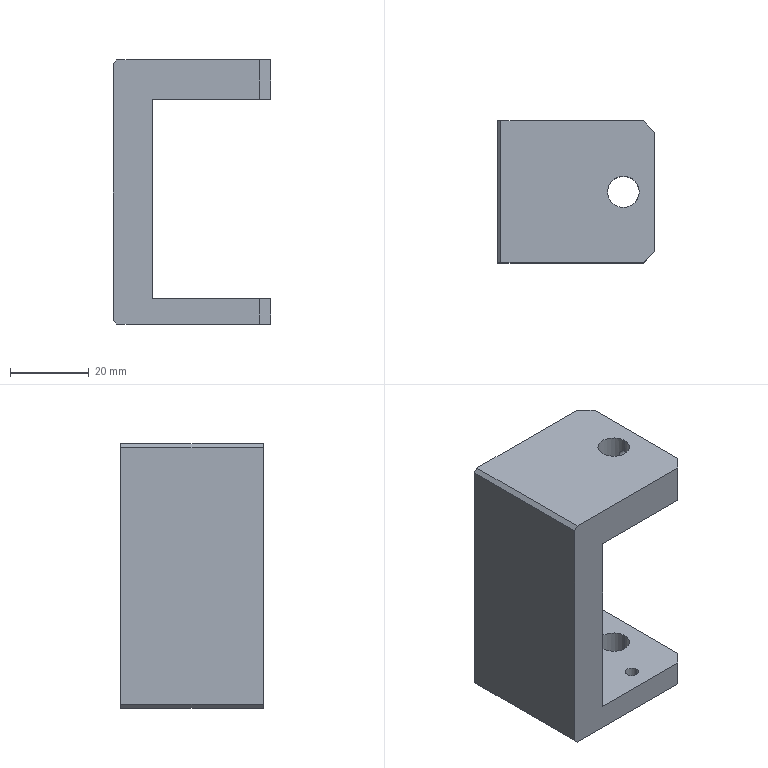Component | SolidWorks | 170423A4-ConveyorBeltIdlerAssembly1-1_170423A4-ConveyorBeltIdlerFixture1-1 | 1 solid | 34 faces | box 40 x 36 x 67 mm | volume 40578 mm3 | plane 16 | cylinder 14 | cone 4 | commonest cylinder face diameters 3.3 x10 8 x4
STEP:
#1=CARTESIAN_POINT('',(0.7383,-3.771,18.844));
#2=VERTEX_POINT('',#1);
#3=CARTESIAN_POINT('',(0.7383,-3.771,18.715));
#4=VERTEX_POINT('',#3);
#5=CARTESIAN_POINT('',(0.7383,-3.771,18.844));
#6=CARTESIAN_POINT('',(0.7383,-3.775,18.844));
#7=CARTESIAN_POINT('',(0.7382,-3.78,18.844));
#8=CARTESIAN_POINT('',(0.7375,-3.788,18.842));
#9=CARTESIAN_POINT('',(0.737,-3.792,18.841));
#10=CARTESIAN_POINT('',(0.7351,-3.804,18.836));
#11=CARTESIAN_POINT('',(0.7333,-3.811,18.831));
#12=CARTESIAN_POINT('',(0.7306,-3.82,18.822));
#13=CARTESIAN_POINT('',(0.7297,-3.823,18.819));
#14=CARTESIAN_POINT('',(0.7279,-3.827,18.812));
#15=CARTESIAN_POINT('',(0.7271,-3.83,18.808));
#16=CARTESIAN_POINT('',(0.7258,-3.833,18.801));
#17=CARTESIAN_POINT('',(0.7253,-3.834,18.797));
#18=CARTESIAN_POINT('',(0.7245,-3.836,18.788));
#19=CARTESIAN_POINT('',(0.7243,-3.836,18.784));
#20=CARTESIAN_POINT('',(0.7243,-3.836,18.771));
#21=CARTESIAN_POINT('',(0.7251,-3.834,18.762));
#22=CARTESIAN_POINT('',(0.7271,-3.83,18.751));
#23=CARTESIAN_POINT('',(0.7279,-3.827,18.747));
#24=CARTESIAN_POINT('',(0.7297,-3.823,18.74));
#25=CARTESIAN_POINT('',(0.7306,-3.82,18.737));
#26=CARTESIAN_POINT('',(0.7324,-3.814,18.731));
#27=CARTESIAN_POINT('',(0.7333,-3.811,18.728));
#28=CARTESIAN_POINT('',(0.7349,-3.804,18.723));
#29=CARTESIAN_POINT('',(0.7357,-3.8,18.721));
#30=CARTESIAN_POINT('',(0.7376,-3.788,18.716));
#31=CARTESIAN_POINT('',(0.7383,-3.78,18.715));
#32=CARTESIAN_POINT('',(0.7383,-3.771,18.715));
#33=B_SPLINE_CURVE_WITH_KNOTS('',3,(#5,#6,#7,#8,#9,#10,#11,#12,#13,#14,#15,#16,#17,#18,#19,#20,#21,#22,#23,#24,#25,#26,#27,#28,#29,#30,#31,#32),.UNSPECIFIED.,.F.,.F.,(4,2,2,2,2,2,2,2,2,2,2,2,2,4),(0.005218,0.005543,0.005869,0.006521,0.006847,0.007173,0.007499,0.007824,0.008476,0.008802,0.009128,0.009454,0.009779,0.01043),.UNSPECIFIED.);
#34=EDGE_CURVE('',#2,#4,#33,.T.);
#35=ORIENTED_EDGE('',*,*,#34,.F.);
#36=CARTESIAN_POINT('',(0.8958,-3.771,18.844));
#37=VERTEX_POINT('',#36);
#38=CARTESIAN_POINT('',(0.8958,-3.771,18.844));
#39=DIRECTION('',(1.,0.,0.));
#40=VECTOR('',#39,39.37);
#41=LINE('',#38,#40);
#42=EDGE_CURVE('',#2,#37,#41,.T.);
#43=ORIENTED_EDGE('',*,*,#42,.T.);
#44=CARTESIAN_POINT('',(0.8958,-3.771,18.715));
#45=VERTEX_POINT('',#44);
#46=CARTESIAN_POINT('',(0.8958,-3.771,18.78));
#47=DIRECTION('',(1.,0.,0.));
#48=DIRECTION('',(0.,0.,-1.));
#49=AXIS2_PLACEMENT_3D('',#46,#47,#48);
#50=CIRCLE('',#49,0.06496);
#51=EDGE_CURVE('',#37,#45,#50,.T.);
#52=ORIENTED_EDGE('',*,*,#51,.T.);
#53=CARTESIAN_POINT('',(0.8958,-3.771,18.715));
#54=DIRECTION('',(1.,0.,0.));
#55=VECTOR('',#54,39.37);
#56=LINE('',#53,#55);
#57=EDGE_CURVE('',#4,#45,#56,.T.);
#58=ORIENTED_EDGE('',*,*,#57,.F.);
#59=EDGE_LOOP('',(#35,#43,#52,#58));
#60=FACE_OUTER_BOUND('',#59,.T.);
#61=CARTESIAN_POINT('',(0.8958,-3.771,18.78));
#62=DIRECTION('',(1.,0.,0.));
#63=DIRECTION('',(0.,0.,-1.));
#64=AXIS2_PLACEMENT_3D('',#61,#62,#63);
#65=CYLINDRICAL_SURFACE('',#64,0.06496);
#66=ADVANCED_FACE('',(#60),#65,.F.);
#67=CARTESIAN_POINT('',(0.2797,-3.279,16.594));
#68=VERTEX_POINT('',#67);
#69=CARTESIAN_POINT('',(0.4096,-3.279,16.594));
#70=VERTEX_POINT('',#69);
#71=CARTESIAN_POINT('',(0.3446,-3.279,16.594));
#72=DIRECTION('',(0.,0.,1.));
#73=DIRECTION('',(-1.,0.,0.));
#74=AXIS2_PLACEMENT_3D('',#71,#72,#73);
#75=CIRCLE('',#74,0.06496);
#76=EDGE_CURVE('',#68,#70,#75,.T.);
#77=ORIENTED_EDGE('',*,*,#76,.T.);
#78=CARTESIAN_POINT('',(0.4096,-3.279,16.339));
#79=VERTEX_POINT('',#78);
#80=CARTESIAN_POINT('',(0.4096,-3.279,16.339));
#81=DIRECTION('',(0.,0.,-1.));
#82=VECTOR('',#81,39.37);
#83=LINE('',#80,#82);
#84=EDGE_CURVE('',#70,#79,#83,.T.);
#85=ORIENTED_EDGE('',*,*,#84,.T.);
#86=CARTESIAN_POINT('',(0.2797,-3.279,16.339));
#87=VERTEX_POINT('',#86);
#88=CARTESIAN_POINT('',(0.3446,-3.279,16.339));
#89=DIRECTION('',(0.,0.,-1.));
#90=DIRECTION('',(-1.,0.,0.));
#91=AXIS2_PLACEMENT_3D('',#88,#89,#90);
#92=CIRCLE('',#91,0.06496);
#93=EDGE_CURVE('',#79,#87,#92,.T.);
#94=ORIENTED_EDGE('',*,*,#93,.T.);
#95=CARTESIAN_POINT('',(0.2797,-3.279,16.339));
#96=DIRECTION('',(0.,0.,-1.));
#97=VECTOR('',#96,39.37);
#98=LINE('',#95,#97);
#99=EDGE_CURVE('',#68,#87,#98,.T.);
#100=ORIENTED_EDGE('',*,*,#99,.F.);
#101=EDGE_LOOP('',(#77,#85,#94,#100));
#102=FACE_OUTER_BOUND('',#101,.T.);
#103=CARTESIAN_POINT('',(0.3446,-3.279,16.339));
#104=DIRECTION('',(0.,0.,-1.));
#105=DIRECTION('',(-1.,0.,0.));
#106=AXIS2_PLACEMENT_3D('',#103,#104,#105);
#107=CYLINDRICAL_SURFACE('',#106,0.06496);
#108=ADVANCED_FACE('',(#102),#107,.F.);
#109=CARTESIAN_POINT('',(0.2797,-4.263,16.594));
#110=VERTEX_POINT('',#109);
#111=CARTESIAN_POINT('',(0.4096,-4.263,16.594));
#112=VERTEX_POINT('',#111);
#113=CARTESIAN_POINT('',(0.3446,-4.263,16.594));
#114=DIRECTION('',(0.,0.,1.));
#115=DIRECTION('',(-1.,0.,0.));
#116=AXIS2_PLACEMENT_3D('',#113,#114,#115);
#117=CIRCLE('',#116,0.06496);
#118=EDGE_CURVE('',#110,#112,#117,.T.);
#119=ORIENTED_EDGE('',*,*,#118,.T.);
#120=CARTESIAN_POINT('',(0.4096,-4.263,16.339));
#121=VERTEX_POINT('',#120);
#122=CARTESIAN_POINT('',(0.4096,-4.263,16.339));
#123=DIRECTION('',(0.,0.,-1.));
#124=VECTOR('',#123,39.37);
#125=LINE('',#122,#124);
#126=EDGE_CURVE('',#112,#121,#125,.T.);
#127=ORIENTED_EDGE('',*,*,#126,.T.);
#128=CARTESIAN_POINT('',(0.2797,-4.263,16.339));
#129=VERTEX_POINT('',#128);
#130=CARTESIAN_POINT('',(0.3446,-4.263,16.339));
#131=DIRECTION('',(0.,0.,-1.));
#132=DIRECTION('',(-1.,0.,0.));
#133=AXIS2_PLACEMENT_3D('',#130,#131,#132);
#134=CIRCLE('',#133,0.06496);
#135=EDGE_CURVE('',#121,#129,#134,.T.);
#136=ORIENTED_EDGE('',*,*,#135,.T.);
#137=CARTESIAN_POINT('',(0.2797,-4.263,16.339));
#138=DIRECTION('',(0.,0.,-1.));
#139=VECTOR('',#138,39.37);
#140=LINE('',#137,#139);
#141=EDGE_CURVE('',#110,#129,#140,.T.);
#142=ORIENTED_EDGE('',*,*,#141,.F.);
#143=EDGE_LOOP('',(#119,#127,#136,#142));
#144=FACE_OUTER_BOUND('',#143,.T.);
#145=CARTESIAN_POINT('',(0.3446,-4.263,16.339));
#146=DIRECTION('',(0.,0.,-1.));
#147=DIRECTION('',(-1.,0.,0.));
#148=AXIS2_PLACEMENT_3D('',#145,#146,#147);
#149=CYLINDRICAL_SURFACE('',#148,0.06496);
#150=ADVANCED_FACE('',(#144),#149,.F.);
#151=CARTESIAN_POINT('',(-0.3778,-3.279,16.791));
#152=VERTEX_POINT('',#151);
#153=CARTESIAN_POINT('',(-0.5077,-3.279,16.791));
#154=VERTEX_POINT('',#153);
#155=CARTESIAN_POINT('',(-0.4428,-3.279,16.791));
#156=DIRECTION('',(0.,0.,-1.));
#157=DIRECTION('',(-1.,0.,0.));
#158=AXIS2_PLACEMENT_3D('',#155,#156,#157);
#159=CIRCLE('',#158,0.06496);
#160=EDGE_CURVE('',#152,#154,#159,.T.);
#161=ORIENTED_EDGE('',*,*,#160,.F.);
#162=CARTESIAN_POINT('',(-0.3778,-3.279,16.339));
#163=VERTEX_POINT('',#162);
#164=CARTESIAN_POINT('',(-0.3778,-3.279,16.339));
#165=DIRECTION('',(0.,0.,-1.));
#166=VECTOR('',#165,39.37);
#167=LINE('',#164,#166);
#168=EDGE_CURVE('',#152,#163,#167,.T.);
#169=ORIENTED_EDGE('',*,*,#168,.T.);
#170=CARTESIAN_POINT('',(-0.5077,-3.279,16.339));
#171=VERTEX_POINT('',#170);
#172=CARTESIAN_POINT('',(-0.4428,-3.279,16.339));
#173=DIRECTION('',(0.,0.,-1.));
#174=DIRECTION('',(-1.,0.,0.));
#175=AXIS2_PLACEMENT_3D('',#172,#173,#174);
#176=CIRCLE('',#175,0.06496);
#177=EDGE_CURVE('',#163,#171,#176,.T.);
#178=ORIENTED_EDGE('',*,*,#177,.T.);
#179=CARTESIAN_POINT('',(-0.5077,-3.279,16.339));
#180=DIRECTION('',(0.,0.,-1.));
#181=VECTOR('',#180,39.37);
#182=LINE('',#179,#181);
#183=EDGE_CURVE('',#154,#171,#182,.T.);
#184=ORIENTED_EDGE('',*,*,#183,.F.);
#185=EDGE_LOOP('',(#161,#169,#178,#184));
#186=FACE_OUTER_BOUND('',#185,.T.);
#187=CARTESIAN_POINT('',(-0.4428,-3.279,16.339));
#188=DIRECTION('',(0.,0.,-1.));
#189=DIRECTION('',(-1.,0.,0.));
#190=AXIS2_PLACEMENT_3D('',#187,#188,#189);
#191=CYLINDRICAL_SURFACE('',#190,0.06496);
#192=ADVANCED_FACE('',(#186),#191,.F.);
#193=CARTESIAN_POINT('',(-0.4428,-3.279,16.83));
#194=VERTEX_POINT('',#193);
#195=CARTESIAN_POINT('',(-0.5077,-3.279,16.791));
#196=DIRECTION('',(-0.8572,0.,-0.515));
#197=VECTOR('',#196,39.37);
#198=LINE('',#195,#197);
#199=EDGE_CURVE('',#194,#154,#198,.T.);
#200=ORIENTED_EDGE('',*,*,#199,.F.);
#201=CARTESIAN_POINT('',(-0.3778,-3.279,16.791));
#202=DIRECTION('',(0.8572,0.,-0.515));
#203=VECTOR('',#202,39.37);
#204=LINE('',#201,#203);
#205=EDGE_CURVE('',#194,#152,#204,.T.);
#206=ORIENTED_EDGE('',*,*,#205,.T.);
#207=ORIENTED_EDGE('',*,*,#160,.T.);
#208=EDGE_LOOP('',(#200,#206,#207));
#209=FACE_OUTER_BOUND('',#208,.T.);
#210=CARTESIAN_POINT('',(-0.4428,-3.279,16.791));
#211=DIRECTION('',(0.,0.,-1.));
#212=DIRECTION('',(-1.,0.,0.));
#213=AXIS2_PLACEMENT_3D('',#210,#211,#212);
#214=CONICAL_SURFACE('',#213,0.06496,1.03);
#215=ADVANCED_FACE('',(#209),#214,.F.);
#216=CARTESIAN_POINT('',(-0.3778,-4.263,16.791));
#217=VERTEX_POINT('',#216);
#218=CARTESIAN_POINT('',(-0.5077,-4.263,16.791));
#219=VERTEX_POINT('',#218);
#220=CARTESIAN_POINT('',(-0.4428,-4.263,16.791));
#221=DIRECTION('',(0.,0.,-1.));
#222=DIRECTION('',(-1.,0.,0.));
#223=AXIS2_PLACEMENT_3D('',#220,#221,#222);
#224=CIRCLE('',#223,0.06496);
#225=EDGE_CURVE('',#217,#219,#224,.T.);
#226=ORIENTED_EDGE('',*,*,#225,.F.);
#227=CARTESIAN_POINT('',(-0.3778,-4.263,16.339));
#228=VERTEX_POINT('',#227);
#229=CARTESIAN_POINT('',(-0.3778,-4.263,16.339));
#230=DIRECTION('',(0.,0.,-1.));
#231=VECTOR('',#230,39.37);
#232=LINE('',#229,#231);
#233=EDGE_CURVE('',#217,#228,#232,.T.);
#234=ORIENTED_EDGE('',*,*,#233,.T.);
#235=CARTESIAN_POINT('',(-0.5077,-4.263,16.339));
#236=VERTEX_POINT('',#235);
#237=CARTESIAN_POINT('',(-0.4428,-4.263,16.339));
#238=DIRECTION('',(0.,0.,-1.));
#239=DIRECTION('',(-1.,0.,0.));
#240=AXIS2_PLACEMENT_3D('',#237,#238,#239);
#241=CIRCLE('',#240,0.06496);
#242=EDGE_CURVE('',#228,#236,#241,.T.);
#243=ORIENTED_EDGE('',*,*,#242,.T.);
#244=CARTESIAN_POINT('',(-0.5077,-4.263,16.339));
#245=DIRECTION('',(0.,0.,-1.));
#246=VECTOR('',#245,39.37);
#247=LINE('',#244,#246);
#248=EDGE_CURVE('',#219,#236,#247,.T.);
#249=ORIENTED_EDGE('',*,*,#248,.F.);
#250=EDGE_LOOP('',(#226,#234,#243,#249));
#251=FACE_OUTER_BOUND('',#250,.T.);
#252=CARTESIAN_POINT('',(-0.4428,-4.263,16.339));
#253=DIRECTION('',(0.,0.,-1.));
#254=DIRECTION('',(-1.,0.,0.));
#255=AXIS2_PLACEMENT_3D('',#252,#253,#254);
#256=CYLINDRICAL_SURFACE('',#255,0.06496);
#257=ADVANCED_FACE('',(#251),#256,.F.);
#258=CARTESIAN_POINT('',(-0.4428,-4.263,16.83));
#259=VERTEX_POINT('',#258);
#260=CARTESIAN_POINT('',(-0.5077,-4.263,16.791));
#261=DIRECTION('',(-0.8572,0.,-0.515));
#262=VECTOR('',#261,39.37);
#263=LINE('',#260,#262);
#264=EDGE_CURVE('',#259,#219,#263,.T.);
#265=ORIENTED_EDGE('',*,*,#264,.F.);
#266=CARTESIAN_POINT('',(-0.3778,-4.263,16.791));
#267=DIRECTION('',(0.8572,0.,-0.515));
#268=VECTOR('',#267,39.37);
#269=LINE('',#266,#268);
#270=EDGE_CURVE('',#259,#217,#269,.T.);
#271=ORIENTED_EDGE('',*,*,#270,.T.);
#272=ORIENTED_EDGE('',*,*,#225,.T.);
#273=EDGE_LOOP('',(#265,#271,#272));
#274=FACE_OUTER_BOUND('',#273,.T.);
#275=CARTESIAN_POINT('',(-0.4428,-4.263,16.791));
#276=DIRECTION('',(0.,0.,-1.));
#277=DIRECTION('',(-1.,0.,0.));
#278=AXIS2_PLACEMENT_3D('',#275,#276,#277);
#279=CONICAL_SURFACE('',#278,0.06496,1.03);
#280=ADVANCED_FACE('',(#274),#279,.F.);
#281=CARTESIAN_POINT('',(0.4234,-3.771,16.339));
#282=VERTEX_POINT('',#281);
#283=CARTESIAN_POINT('',(0.7383,-3.771,16.339));
#284=VERTEX_POINT('',#283);
#285=CARTESIAN_POINT('',(0.5808,-3.771,16.339));
#286=DIRECTION('',(0.,0.,1.));
#287=DIRECTION('',(1.,0.,0.));
#288=AXIS2_PLACEMENT_3D('',#285,#286,#287);
#289=CIRCLE('',#288,0.1575);
#290=EDGE_CURVE('',#282,#284,#289,.T.);
#291=ORIENTED_EDGE('',*,*,#290,.F.);
#292=CARTESIAN_POINT('',(0.4234,-3.771,16.594));
#293=VERTEX_POINT('',#292);
#294=CARTESIAN_POINT('',(0.4234,-3.771,18.976));
#295=DIRECTION('',(0.,0.,1.));
#296=VECTOR('',#295,39.37);
#297=LINE('',#294,#296);
#298=EDGE_CURVE('',#282,#293,#297,.T.);
#299=ORIENTED_EDGE('',*,*,#298,.T.);
#300=CARTESIAN_POINT('',(0.7383,-3.771,16.594));
#301=VERTEX_POINT('',#300);
#302=CARTESIAN_POINT('',(0.5808,-3.771,16.594));
#303=DIRECTION('',(0.,0.,1.));
#304=DIRECTION('',(-1.,0.,0.));
#305=AXIS2_PLACEMENT_3D('',#302,#303,#304);
#306=CIRCLE('',#305,0.1575);
#307=EDGE_CURVE('',#293,#301,#306,.T.);
#308=ORIENTED_EDGE('',*,*,#307,.T.);
#309=CARTESIAN_POINT('',(0.7383,-3.771,18.976));
#310=DIRECTION('',(0.,0.,1.));
#311=VECTOR('',#310,39.37);
#312=LINE('',#309,#311);
#313=EDGE_CURVE('',#284,#301,#312,.T.);
#314=ORIENTED_EDGE('',*,*,#313,.F.);
#315=EDGE_LOOP('',(#291,#299,#308,#314));
#316=FACE_OUTER_BOUND('',#315,.T.);
#317=CARTESIAN_POINT('',(0.5808,-3.771,18.976));
#318=DIRECTION('',(0.,0.,1.));
#319=DIRECTION('',(1.,0.,0.));
#320=AXIS2_PLACEMENT_3D('',#317,#318,#319);
#321=CYLINDRICAL_SURFACE('',#320,0.1575);
#322=ADVANCED_FACE('',(#316),#321,.F.);
#323=CARTESIAN_POINT('',(0.7383,-3.771,18.583));
#324=VERTEX_POINT('',#323);
#325=CARTESIAN_POINT('',(0.4234,-3.771,18.583));
#326=VERTEX_POINT('',#325);
#327=CARTESIAN_POINT('',(0.5808,-3.771,18.583));
#328=DIRECTION('',(-0.,0.,-1.));
#329=DIRECTION('',(1.,0.,0.));
#330=AXIS2_PLACEMENT_3D('',#327,#328,#329);
#331=CIRCLE('',#330,0.1575);
#332=EDGE_CURVE('',#324,#326,#331,.T.);
#333=ORIENTED_EDGE('',*,*,#332,.T.);
#334=CARTESIAN_POINT('',(0.4234,-3.771,18.976));
#335=VERTEX_POINT('',#334);
#336=CARTESIAN_POINT('',(0.4234,-3.771,18.976));
#337=DIRECTION('',(0.,0.,1.));
#338=VECTOR('',#337,39.37);
#339=LINE('',#336,#338);
#340=EDGE_CURVE('',#326,#335,#339,.T.);
#341=ORIENTED_EDGE('',*,*,#340,.T.);
#342=CARTESIAN_POINT('',(0.7383,-3.771,18.976));
#343=VERTEX_POINT('',#342);
#344=CARTESIAN_POINT('',(0.5808,-3.771,18.976));
#345=DIRECTION('',(0.,0.,1.));
#346=DIRECTION('',(1.,0.,0.));
#347=AXIS2_PLACEMENT_3D('',#344,#345,#346);
#348=CIRCLE('',#347,0.1575);
#349=EDGE_CURVE('',#335,#343,#348,.T.);
#350=ORIENTED_EDGE('',*,*,#349,.T.);
#351=CARTESIAN_POINT('',(0.7383,-3.771,18.976));
#352=DIRECTION('',(0.,0.,1.));
#353=VECTOR('',#352,39.37);
#354=LINE('',#351,#353);
#355=EDGE_CURVE('',#2,#343,#354,.T.);
#356=ORIENTED_EDGE('',*,*,#355,.F.);
#357=ORIENTED_EDGE('',*,*,#34,.T.);
#358=CARTESIAN_POINT('',(0.7383,-3.771,18.976));
#359=DIRECTION('',(0.,0.,1.));
#360=VECTOR('',#359,39.37);
#361=LINE('',#358,#360);
#362=EDGE_CURVE('',#324,#4,#361,.T.);
#363=ORIENTED_EDGE('',*,*,#362,.F.);
#364=EDGE_LOOP('',(#333,#341,#350,#356,#357,#363));
#365=FACE_OUTER_BOUND('',#364,.T.);
#366=CARTESIAN_POINT('',(0.5808,-3.771,18.976));
#367=DIRECTION('',(0.,0.,1.));
#368=DIRECTION('',(1.,0.,0.));
#369=AXIS2_PLACEMENT_3D('',#366,#367,#368);
#370=CYLINDRICAL_SURFACE('',#369,0.1575);
#371=ADVANCED_FACE('',(#365),#370,.F.);
#372=CARTESIAN_POINT('',(0.8958,-3.771,18.78));
#373=DIRECTION('',(1.,0.,0.));
#374=DIRECTION('',(0.,0.,-1.));
#375=AXIS2_PLACEMENT_3D('',#372,#373,#374);
#376=CIRCLE('',#375,0.06496);
#377=EDGE_CURVE('',#45,#37,#376,.T.);
#378=ORIENTED_EDGE('',*,*,#377,.F.);
#379=ORIENTED_EDGE('',*,*,#51,.F.);
#380=EDGE_LOOP('',(#378,#379));
#381=FACE_BOUND('',#380,.T.);
#382=CARTESIAN_POINT('',(0.8958,-4.362,18.976));
#383=VERTEX_POINT('',#382);
#384=CARTESIAN_POINT('',(0.8958,-3.181,18.976));
#385=VERTEX_POINT('',#384);
#386=CARTESIAN_POINT('',(0.8958,-4.48,18.976));
#387=DIRECTION('',(0.,1.,0.));
#388=VECTOR('',#387,39.37);
#389=LINE('',#386,#388);
#390=EDGE_CURVE('',#383,#385,#389,.T.);
#391=ORIENTED_EDGE('',*,*,#390,.F.);
#392=CARTESIAN_POINT('',(0.8958,-4.362,18.583));
#393=VERTEX_POINT('',#392);
#394=CARTESIAN_POINT('',(0.8958,-4.362,18.976));
#395=DIRECTION('',(0.,0.,-1.));
#396=VECTOR('',#395,39.37);
#397=LINE('',#394,#396);
#398=EDGE_CURVE('',#383,#393,#397,.T.);
#399=ORIENTED_EDGE('',*,*,#398,.T.);
#400=CARTESIAN_POINT('',(0.8958,-3.181,18.583));
#401=VERTEX_POINT('',#400);
#402=CARTESIAN_POINT('',(0.8958,-4.48,18.583));
#403=DIRECTION('',(0.,1.,0.));
#404=VECTOR('',#403,39.37);
#405=LINE('',#402,#404);
#406=EDGE_CURVE('',#393,#401,#405,.T.);
#407=ORIENTED_EDGE('',*,*,#406,.T.);
#408=CARTESIAN_POINT('',(0.8958,-3.181,18.976));
#409=DIRECTION('',(0.,0.,1.));
#410=VECTOR('',#409,39.37);
#411=LINE('',#408,#410);
#412=EDGE_CURVE('',#401,#385,#411,.T.);
#413=ORIENTED_EDGE('',*,*,#412,.T.);
#414=EDGE_LOOP('',(#391,#399,#407,#413));
#415=FACE_OUTER_BOUND('',#414,.T.);
#416=CARTESIAN_POINT('',(0.8958,-4.48,18.976));
#417=DIRECTION('',(-1.,0.,0.));
#418=DIRECTION('',(0.,0.,1.));
#419=AXIS2_PLACEMENT_3D('',#416,#417,#418);
#420=PLANE('',#419);
#421=ADVANCED_FACE('',(#381,#415),#420,.F.);
#422=ORIENTED_EDGE('',*,*,#340,.F.);
#423=CARTESIAN_POINT('',(0.5808,-3.771,18.583));
#424=DIRECTION('',(-0.,0.,-1.));
#425=DIRECTION('',(1.,0.,0.));
#426=AXIS2_PLACEMENT_3D('',#423,#424,#425);
#427=CIRCLE('',#426,0.1575);
#428=EDGE_CURVE('',#326,#324,#427,.T.);
#429=ORIENTED_EDGE('',*,*,#428,.T.);
#430=ORIENTED_EDGE('',*,*,#362,.T.);
#431=CARTESIAN_POINT('',(0.7383,-3.771,18.715));
#432=CARTESIAN_POINT('',(0.7383,-3.767,18.715));
#433=CARTESIAN_POINT('',(0.7382,-3.763,18.715));
#434=CARTESIAN_POINT('',(0.7375,-3.754,18.717));
#435=CARTESIAN_POINT('',(0.737,-3.75,18.718));
#436=CARTESIAN_POINT('',(0.7351,-3.738,18.723));
#437=CARTESIAN_POINT('',(0.7333,-3.731,18.728));
#438=CARTESIAN_POINT('',(0.7297,-3.719,18.74));
#439=CARTESIAN_POINT('',(0.7278,-3.715,18.747));
#440=CARTESIAN_POINT('',(0.7258,-3.71,18.758));
#441=CARTESIAN_POINT('',(0.7252,-3.708,18.763));
#442=CARTESIAN_POINT('',(0.7245,-3.707,18.771));
#443=CARTESIAN_POINT('',(0.7243,-3.706,18.775));
#444=CARTESIAN_POINT('',(0.7243,-3.706,18.784));
#445=CARTESIAN_POINT('',(0.7245,-3.707,18.788));
#446=CARTESIAN_POINT('',(0.7252,-3.708,18.797));
#447=CARTESIAN_POINT('',(0.7258,-3.71,18.801));
#448=CARTESIAN_POINT('',(0.7272,-3.713,18.809));
#449=CARTESIAN_POINT('',(0.7279,-3.715,18.812));
#450=CARTESIAN_POINT('',(0.7297,-3.72,18.819));
#451=CARTESIAN_POINT('',(0.7306,-3.722,18.823));
#452=CARTESIAN_POINT('',(0.7324,-3.728,18.828));
#453=CARTESIAN_POINT('',(0.7333,-3.731,18.831));
#454=CARTESIAN_POINT('',(0.7349,-3.739,18.836));
#455=CARTESIAN_POINT('',(0.7357,-3.742,18.838));
#456=CARTESIAN_POINT('',(0.7376,-3.754,18.843));
#457=CARTESIAN_POINT('',(0.7383,-3.763,18.844));
#458=CARTESIAN_POINT('',(0.7383,-3.771,18.844));
#459=B_SPLINE_CURVE_WITH_KNOTS('',3,(#431,#432,#433,#434,#435,#436,#437,#438,#439,#440,#441,#442,#443,#444,#445,#446,#447,#448,#449,#450,#451,#452,#453,#454,#455,#456,#457,#458),.UNSPECIFIED.,.F.,.F.,(4,2,2,2,2,2,2,2,2,2,2,2,2,4),(0.,0.0003261,0.0006522,0.001304,0.001957,0.002283,0.002609,0.002935,0.003261,0.003587,0.003913,0.004239,0.004565,0.005218),.UNSPECIFIED.);
#460=EDGE_CURVE('',#4,#2,#459,.T.);
#461=ORIENTED_EDGE('',*,*,#460,.T.);
#462=ORIENTED_EDGE('',*,*,#355,.T.);
#463=CARTESIAN_POINT('',(0.5808,-3.771,18.976));
#464=DIRECTION('',(0.,0.,1.));
#465=DIRECTION('',(1.,0.,0.));
#466=AXIS2_PLACEMENT_3D('',#463,#464,#465);
#467=CIRCLE('',#466,0.1575);
#468=EDGE_CURVE('',#343,#335,#467,.T.);
#469=ORIENTED_EDGE('',*,*,#468,.T.);
#470=EDGE_LOOP('',(#422,#429,#430,#461,#462,#469));
#471=FACE_OUTER_BOUND('',#470,.T.);
#472=CARTESIAN_POINT('',(0.5808,-3.771,18.976));
#473=DIRECTION('',(0.,0.,1.));
#474=DIRECTION('',(1.,0.,0.));
#475=AXIS2_PLACEMENT_3D('',#472,#473,#474);
#476=CYLINDRICAL_SURFACE('',#475,0.1575);
#477=ADVANCED_FACE('',(#471),#476,.F.);
#478=CARTESIAN_POINT('',(-0.679,-3.063,18.937));
#479=VERTEX_POINT('',#478);
#480=CARTESIAN_POINT('',(-0.679,-3.063,16.378));
#481=VERTEX_POINT('',#480);
#482=CARTESIAN_POINT('',(-0.679,-3.063,18.976));
#483=DIRECTION('',(0.,0.,-1.));
#484=VECTOR('',#483,39.37);
#485=LINE('',#482,#484);
#486=EDGE_CURVE('',#479,#481,#485,.T.);
#487=ORIENTED_EDGE('',*,*,#486,.T.);
#488=CARTESIAN_POINT('',(-0.679,-4.48,16.378));
#489=VERTEX_POINT('',#488);
#490=CARTESIAN_POINT('',(-0.679,-4.48,16.378));
#491=DIRECTION('',(0.,-1.,0.));
#492=VECTOR('',#491,39.37);
#493=LINE('',#490,#492);
#494=EDGE_CURVE('',#481,#489,#493,.T.);
#495=ORIENTED_EDGE('',*,*,#494,.T.);
#496=CARTESIAN_POINT('',(-0.679,-4.48,18.937));
#497=VERTEX_POINT('',#496);
#498=CARTESIAN_POINT('',(-0.679,-4.48,18.976));
#499=DIRECTION('',(0.,0.,-1.));
#500=VECTOR('',#499,39.37);
#501=LINE('',#498,#500);
#502=EDGE_CURVE('',#497,#489,#501,.T.);
#503=ORIENTED_EDGE('',*,*,#502,.F.);
#504=CARTESIAN_POINT('',(-0.679,-4.48,18.937));
#505=DIRECTION('',(0.,1.,0.));
#506=VECTOR('',#505,39.37);
#507=LINE('',#504,#506);
#508=EDGE_CURVE('',#497,#479,#507,.T.);
#509=ORIENTED_EDGE('',*,*,#508,.T.);
#510=EDGE_LOOP('',(#487,#495,#503,#509));
#511=FACE_OUTER_BOUND('',#510,.T.);
#512=CARTESIAN_POINT('',(-0.679,-4.48,18.976));
#513=DIRECTION('',(1.,0.,0.));
#514=DIRECTION('',(0.,0.,-1.));
#515=AXIS2_PLACEMENT_3D('',#512,#513,#514);
#516=PLANE('',#515);
#517=ADVANCED_FACE('',(#511),#516,.F.);
#518=ORIENTED_EDGE('',*,*,#502,.T.);
#519=CARTESIAN_POINT('',(-0.6396,-4.48,16.339));
#520=VERTEX_POINT('',#519);
#521=CARTESIAN_POINT('',(-0.679,-4.48,16.378));
#522=DIRECTION('',(0.7071,0.,-0.7071));
#523=VECTOR('',#522,39.37);
#524=LINE('',#521,#523);
#525=EDGE_CURVE('',#489,#520,#524,.T.);
#526=ORIENTED_EDGE('',*,*,#525,.T.);
#527=CARTESIAN_POINT('',(0.7777,-4.48,16.339));
#528=VERTEX_POINT('',#527);
#529=CARTESIAN_POINT('',(-0.679,-4.48,16.339));
#530=DIRECTION('',(1.,0.,0.));
#531=VECTOR('',#530,39.37);
#532=LINE('',#529,#531);
#533=EDGE_CURVE('',#520,#528,#532,.T.);
#534=ORIENTED_EDGE('',*,*,#533,.T.);
#535=CARTESIAN_POINT('',(0.7777,-4.48,16.594));
#536=VERTEX_POINT('',#535);
#537=CARTESIAN_POINT('',(0.7777,-4.48,18.976));
#538=DIRECTION('',(0.,0.,1.));
#539=VECTOR('',#538,39.37);
#540=LINE('',#537,#539);
#541=EDGE_CURVE('',#528,#536,#540,.T.);
#542=ORIENTED_EDGE('',*,*,#541,.T.);
#543=CARTESIAN_POINT('',(-0.2853,-4.48,16.594));
#544=VERTEX_POINT('',#543);
#545=CARTESIAN_POINT('',(0.8958,-4.48,16.594));
#546=DIRECTION('',(-1.,0.,0.));
#547=VECTOR('',#546,39.37);
#548=LINE('',#545,#547);
#549=EDGE_CURVE('',#536,#544,#548,.T.);
#550=ORIENTED_EDGE('',*,*,#549,.T.);
#551=CARTESIAN_POINT('',(-0.2853,-4.48,18.583));
#552=VERTEX_POINT('',#551);
#553=CARTESIAN_POINT('',(-0.2853,-4.48,16.594));
#554=DIRECTION('',(0.,0.,1.));
#555=VECTOR('',#554,39.37);
#556=LINE('',#553,#555);
#557=EDGE_CURVE('',#544,#552,#556,.T.);
#558=ORIENTED_EDGE('',*,*,#557,.T.);
#559=CARTESIAN_POINT('',(0.7777,-4.48,18.583));
#560=VERTEX_POINT('',#559);
#561=CARTESIAN_POINT('',(0.8958,-4.48,18.583));
#562=DIRECTION('',(1.,0.,-0.));
#563=VECTOR('',#562,39.37);
#564=LINE('',#561,#563);
#565=EDGE_CURVE('',#552,#560,#564,.T.);
#566=ORIENTED_EDGE('',*,*,#565,.T.);
#567=CARTESIAN_POINT('',(0.7777,-4.48,18.976));
#568=VERTEX_POINT('',#567);
#569=CARTESIAN_POINT('',(0.7777,-4.48,18.976));
#570=DIRECTION('',(0.,0.,1.));
#571=VECTOR('',#570,39.37);
#572=LINE('',#569,#571);
#573=EDGE_CURVE('',#560,#568,#572,.T.);
#574=ORIENTED_EDGE('',*,*,#573,.T.);
#575=CARTESIAN_POINT('',(-0.6396,-4.48,18.976));
#576=VERTEX_POINT('',#575);
#577=CARTESIAN_POINT('',(-0.679,-4.48,18.976));
#578=DIRECTION('',(1.,0.,0.));
#579=VECTOR('',#578,39.37);
#580=LINE('',#577,#579);
#581=EDGE_CURVE('',#576,#568,#580,.T.);
#582=ORIENTED_EDGE('',*,*,#581,.F.);
#583=CARTESIAN_POINT('',(-0.6396,-4.48,18.976));
#584=DIRECTION('',(-0.7071,0.,-0.7071));
#585=VECTOR('',#584,39.37);
#586=LINE('',#583,#585);
#587=EDGE_CURVE('',#576,#497,#586,.T.);
#588=ORIENTED_EDGE('',*,*,#587,.T.);
#589=EDGE_LOOP('',(#518,#526,#534,#542,#550,#558,#566,#574,#582,#588));
#590=FACE_OUTER_BOUND('',#589,.T.);
#591=CARTESIAN_POINT('',(-0.679,-4.48,18.976));
#592=DIRECTION('',(0.,1.,0.));
#593=DIRECTION('',(0.,0.,1.));
#594=AXIS2_PLACEMENT_3D('',#591,#592,#593);
#595=PLANE('',#594);
#596=ADVANCED_FACE('',(#590),#595,.F.);
#597=CARTESIAN_POINT('',(0.8958,-4.362,16.339));
#598=VERTEX_POINT('',#597);
#599=CARTESIAN_POINT('',(0.8958,-3.181,16.339));
#600=VERTEX_POINT('',#599);
#601=CARTESIAN_POINT('',(0.8958,-4.48,16.339));
#602=DIRECTION('',(0.,1.,0.));
#603=VECTOR('',#602,39.37);
#604=LINE('',#601,#603);
#605=EDGE_CURVE('',#598,#600,#604,.T.);
#606=ORIENTED_EDGE('',*,*,#605,.T.);
#607=CARTESIAN_POINT('',(0.8958,-3.181,16.594));
#608=VERTEX_POINT('',#607);
#609=CARTESIAN_POINT('',(0.8958,-3.181,18.976));
#610=DIRECTION('',(0.,0.,1.));
#611=VECTOR('',#610,39.37);
#612=LINE('',#609,#611);
#613=EDGE_CURVE('',#600,#608,#612,.T.);
#614=ORIENTED_EDGE('',*,*,#613,.T.);
#615=CARTESIAN_POINT('',(0.8958,-4.362,16.594));
#616=VERTEX_POINT('',#615);
#617=CARTESIAN_POINT('',(0.8958,-4.48,16.594));
#618=DIRECTION('',(0.,1.,0.));
#619=VECTOR('',#618,39.37);
#620=LINE('',#617,#619);
#621=EDGE_CURVE('',#616,#608,#620,.T.);
#622=ORIENTED_EDGE('',*,*,#621,.F.);
#623=CARTESIAN_POINT('',(0.8958,-4.362,18.976));
#624=DIRECTION('',(0.,0.,-1.));
#625=VECTOR('',#624,39.37);
#626=LINE('',#623,#625);
#627=EDGE_CURVE('',#616,#598,#626,.T.);
#628=ORIENTED_EDGE('',*,*,#627,.T.);
#629=EDGE_LOOP('',(#606,#614,#622,#628));
#630=FACE_OUTER_BOUND('',#629,.T.);
#631=CARTESIAN_POINT('',(0.8958,-4.48,18.976));
#632=DIRECTION('',(-1.,0.,0.));
#633=DIRECTION('',(0.,0.,1.));
#634=AXIS2_PLACEMENT_3D('',#631,#632,#633);
#635=PLANE('',#634);
#636=ADVANCED_FACE('',(#630),#635,.F.);
#637=CARTESIAN_POINT('',(0.7777,-3.063,16.339));
#638=VERTEX_POINT('',#637);
#639=CARTESIAN_POINT('',(-0.6396,-3.063,16.339));
#640=VERTEX_POINT('',#639);
#641=CARTESIAN_POINT('',(-0.679,-3.063,16.339));
#642=DIRECTION('',(-1.,0.,0.));
#643=VECTOR('',#642,39.37);
#644=LINE('',#641,#643);
#645=EDGE_CURVE('',#638,#640,#644,.T.);
#646=ORIENTED_EDGE('',*,*,#645,.T.);
#647=CARTESIAN_POINT('',(-0.679,-3.063,16.378));
#648=DIRECTION('',(-0.7071,0.,0.7071));
#649=VECTOR('',#648,39.37);
#650=LINE('',#647,#649);
#651=EDGE_CURVE('',#640,#481,#650,.T.);
#652=ORIENTED_EDGE('',*,*,#651,.T.);
#653=ORIENTED_EDGE('',*,*,#486,.F.);
#654=CARTESIAN_POINT('',(-0.6396,-3.063,18.976));
#655=VERTEX_POINT('',#654);
#656=CARTESIAN_POINT('',(-0.6396,-3.063,18.976));
#657=DIRECTION('',(0.7071,0.,0.7071));
#658=VECTOR('',#657,39.37);
#659=LINE('',#656,#658);
#660=EDGE_CURVE('',#479,#655,#659,.T.);
#661=ORIENTED_EDGE('',*,*,#660,.T.);
#662=CARTESIAN_POINT('',(0.7777,-3.063,18.976));
#663=VERTEX_POINT('',#662);
#664=CARTESIAN_POINT('',(-0.679,-3.063,18.976));
#665=DIRECTION('',(-1.,0.,0.));
#666=VECTOR('',#665,39.37);
#667=LINE('',#664,#666);
#668=EDGE_CURVE('',#663,#655,#667,.T.);
#669=ORIENTED_EDGE('',*,*,#668,.F.);
#670=CARTESIAN_POINT('',(0.7777,-3.063,18.583));
#671=VERTEX_POINT('',#670);
#672=CARTESIAN_POINT('',(0.7777,-3.063,18.976));
#673=DIRECTION('',(0.,0.,-1.));
#674=VECTOR('',#673,39.37);
#675=LINE('',#672,#674);
#676=EDGE_CURVE('',#663,#671,#675,.T.);
#677=ORIENTED_EDGE('',*,*,#676,.T.);
#678=CARTESIAN_POINT('',(-0.2853,-3.063,18.583));
#679=VERTEX_POINT('',#678);
#680=CARTESIAN_POINT('',(0.8958,-3.063,18.583));
#681=DIRECTION('',(1.,0.,-0.));
#682=VECTOR('',#681,39.37);
#683=LINE('',#680,#682);
#684=EDGE_CURVE('',#679,#671,#683,.T.);
#685=ORIENTED_EDGE('',*,*,#684,.F.);
#686=CARTESIAN_POINT('',(-0.2853,-3.063,16.594));
#687=VERTEX_POINT('',#686);
#688=CARTESIAN_POINT('',(-0.2853,-3.063,16.594));
#689=DIRECTION('',(0.,0.,1.));
#690=VECTOR('',#689,39.37);
#691=LINE('',#688,#690);
#692=EDGE_CURVE('',#687,#679,#691,.T.);
#693=ORIENTED_EDGE('',*,*,#692,.F.);
#694=CARTESIAN_POINT('',(0.7777,-3.063,16.594));
#695=VERTEX_POINT('',#694);
#696=CARTESIAN_POINT('',(0.8958,-3.063,16.594));
#697=DIRECTION('',(-1.,0.,0.));
#698=VECTOR('',#697,39.37);
#699=LINE('',#696,#698);
#700=EDGE_CURVE('',#695,#687,#699,.T.);
#701=ORIENTED_EDGE('',*,*,#700,.F.);
#702=CARTESIAN_POINT('',(0.7777,-3.063,18.976));
#703=DIRECTION('',(0.,0.,-1.));
#704=VECTOR('',#703,39.37);
#705=LINE('',#702,#704);
#706=EDGE_CURVE('',#695,#638,#705,.T.);
#707=ORIENTED_EDGE('',*,*,#706,.T.);
#708=EDGE_LOOP('',(#646,#652,#653,#661,#669,#677,#685,#693,#701,#707));
#709=FACE_OUTER_BOUND('',#708,.T.);
#710=CARTESIAN_POINT('',(-0.679,-3.063,18.976));
#711=DIRECTION('',(0.,-1.,0.));
#712=DIRECTION('',(0.,0.,-1.));
#713=AXIS2_PLACEMENT_3D('',#710,#711,#712);
#714=PLANE('',#713);
#715=ADVANCED_FACE('',(#709),#714,.F.);
#716=ORIENTED_EDGE('',*,*,#468,.F.);
#717=ORIENTED_EDGE('',*,*,#349,.F.);
#718=EDGE_LOOP('',(#716,#717));
#719=FACE_BOUND('',#718,.T.);
#720=ORIENTED_EDGE('',*,*,#668,.T.);
#721=CARTESIAN_POINT('',(-0.6396,-4.48,18.976));
#722=DIRECTION('',(0.,-1.,0.));
#723=VECTOR('',#722,39.37);
#724=LINE('',#721,#723);
#725=EDGE_CURVE('',#655,#576,#724,.T.);
#726=ORIENTED_EDGE('',*,*,#725,.T.);
#727=ORIENTED_EDGE('',*,*,#581,.T.);
#728=CARTESIAN_POINT('',(0.8958,-4.362,18.976));
#729=DIRECTION('',(0.7071,0.7071,0.));
#730=VECTOR('',#729,39.37);
#731=LINE('',#728,#730);
#732=EDGE_CURVE('',#568,#383,#731,.T.);
#733=ORIENTED_EDGE('',*,*,#732,.T.);
#734=ORIENTED_EDGE('',*,*,#390,.T.);
#735=CARTESIAN_POINT('',(0.7777,-3.063,18.976));
#736=DIRECTION('',(-0.7071,0.7071,0.));
#737=VECTOR('',#736,39.37);
#738=LINE('',#735,#737);
#739=EDGE_CURVE('',#385,#663,#738,.T.);
#740=ORIENTED_EDGE('',*,*,#739,.T.);
#741=EDGE_LOOP('',(#720,#726,#727,#733,#734,#740));
#742=FACE_OUTER_BOUND('',#741,.T.);
#743=CARTESIAN_POINT('',(-0.679,-4.48,18.976));
#744=DIRECTION('',(0.,0.,-1.));
#745=DIRECTION('',(-1.,0.,0.));
#746=AXIS2_PLACEMENT_3D('',#743,#744,#745);
#747=PLANE('',#746);
#748=ADVANCED_FACE('',(#719,#742),#747,.F.);
#749=CARTESIAN_POINT('',(0.3446,-3.279,16.339));
#750=DIRECTION('',(0.,0.,-1.));
#751=DIRECTION('',(-1.,0.,0.));
#752=AXIS2_PLACEMENT_3D('',#749,#750,#751);
#753=CIRCLE('',#752,0.06496);
#754=EDGE_CURVE('',#87,#79,#753,.T.);
#755=ORIENTED_EDGE('',*,*,#754,.F.);
#756=ORIENTED_EDGE('',*,*,#93,.F.);
#757=EDGE_LOOP('',(#755,#756));
#758=FACE_BOUND('',#757,.T.);
#759=CARTESIAN_POINT('',(0.3446,-4.263,16.339));
#760=DIRECTION('',(0.,0.,-1.));
#761=DIRECTION('',(-1.,0.,0.));
#762=AXIS2_PLACEMENT_3D('',#759,#760,#761);
#763=CIRCLE('',#762,0.06496);
#764=EDGE_CURVE('',#129,#121,#763,.T.);
#765=ORIENTED_EDGE('',*,*,#764,.F.);
#766=ORIENTED_EDGE('',*,*,#135,.F.);
#767=EDGE_LOOP('',(#765,#766));
#768=FACE_BOUND('',#767,.T.);
#769=CARTESIAN_POINT('',(-0.4428,-3.279,16.339));
#770=DIRECTION('',(0.,0.,-1.));
#771=DIRECTION('',(-1.,0.,0.));
#772=AXIS2_PLACEMENT_3D('',#769,#770,#771);
#773=CIRCLE('',#772,0.06496);
#774=EDGE_CURVE('',#171,#163,#773,.T.);
#775=ORIENTED_EDGE('',*,*,#774,.F.);
#776=ORIENTED_EDGE('',*,*,#177,.F.);
#777=EDGE_LOOP('',(#775,#776));
#778=FACE_BOUND('',#777,.T.);
#779=CARTESIAN_POINT('',(-0.4428,-4.263,16.339));
#780=DIRECTION('',(0.,0.,-1.));
#781=DIRECTION('',(-1.,0.,0.));
#782=AXIS2_PLACEMENT_3D('',#779,#780,#781);
#783=CIRCLE('',#782,0.06496);
#784=EDGE_CURVE('',#236,#228,#783,.T.);
#785=ORIENTED_EDGE('',*,*,#784,.F.);
#786=ORIENTED_EDGE('',*,*,#242,.F.);
#787=EDGE_LOOP('',(#785,#786));
#788=FACE_BOUND('',#787,.T.);
#789=CARTESIAN_POINT('',(0.5808,-3.771,16.339));
#790=DIRECTION('',(0.,0.,1.));
#791=DIRECTION('',(1.,0.,0.));
#792=AXIS2_PLACEMENT_3D('',#789,#790,#791);
#793=CIRCLE('',#792,0.1575);
#794=EDGE_CURVE('',#284,#282,#793,.T.);
#795=ORIENTED_EDGE('',*,*,#794,.T.);
#796=ORIENTED_EDGE('',*,*,#290,.T.);
#797=EDGE_LOOP('',(#795,#796));
#798=FACE_BOUND('',#797,.T.);
#799=ORIENTED_EDGE('',*,*,#533,.F.);
#800=CARTESIAN_POINT('',(-0.6396,-3.063,16.339));
#801=DIRECTION('',(0.,1.,0.));
#802=VECTOR('',#801,39.37);
#803=LINE('',#800,#802);
#804=EDGE_CURVE('',#520,#640,#803,.T.);
#805=ORIENTED_EDGE('',*,*,#804,.T.);
#806=ORIENTED_EDGE('',*,*,#645,.F.);
#807=CARTESIAN_POINT('',(0.758,-3.043,16.339));
#808=DIRECTION('',(0.7071,-0.7071,0.));
#809=VECTOR('',#808,39.37);
#810=LINE('',#807,#809);
#811=EDGE_CURVE('',#638,#600,#810,.T.);
#812=ORIENTED_EDGE('',*,*,#811,.T.);
#813=ORIENTED_EDGE('',*,*,#605,.F.);
#814=CARTESIAN_POINT('',(0.04935,-5.208,16.339));
#815=DIRECTION('',(-0.7071,-0.7071,0.));
#816=VECTOR('',#815,39.37);
#817=LINE('',#814,#816);
#818=EDGE_CURVE('',#598,#528,#817,.T.);
#819=ORIENTED_EDGE('',*,*,#818,.T.);
#820=EDGE_LOOP('',(#799,#805,#806,#812,#813,#819));
#821=FACE_OUTER_BOUND('',#820,.T.);
#822=CARTESIAN_POINT('',(-0.679,-4.48,16.339));
#823=DIRECTION('',(0.,0.,-1.));
#824=DIRECTION('',(-1.,0.,0.));
#825=AXIS2_PLACEMENT_3D('',#822,#823,#824);
#826=PLANE('',#825);
#827=ADVANCED_FACE('',(#758,#768,#778,#788,#798,#821),#826,.T.);
#828=ORIENTED_EDGE('',*,*,#298,.F.);
#829=ORIENTED_EDGE('',*,*,#794,.F.);
#830=ORIENTED_EDGE('',*,*,#313,.T.);
#831=CARTESIAN_POINT('',(0.5808,-3.771,16.594));
#832=DIRECTION('',(0.,0.,1.));
#833=DIRECTION('',(-1.,0.,0.));
#834=AXIS2_PLACEMENT_3D('',#831,#832,#833);
#835=CIRCLE('',#834,0.1575);
#836=EDGE_CURVE('',#301,#293,#835,.T.);
#837=ORIENTED_EDGE('',*,*,#836,.T.);
#838=EDGE_LOOP('',(#828,#829,#830,#837));
#839=FACE_OUTER_BOUND('',#838,.T.);
#840=CARTESIAN_POINT('',(0.5808,-3.771,18.976));
#841=DIRECTION('',(0.,0.,1.));
#842=DIRECTION('',(1.,0.,0.));
#843=AXIS2_PLACEMENT_3D('',#840,#841,#842);
#844=CYLINDRICAL_SURFACE('',#843,0.1575);
#845=ADVANCED_FACE('',(#839),#844,.F.);
#846=ORIENTED_EDGE('',*,*,#270,.F.);
#847=ORIENTED_EDGE('',*,*,#264,.T.);
#848=CARTESIAN_POINT('',(-0.4428,-4.263,16.791));
#849=DIRECTION('',(0.,0.,-1.));
#850=DIRECTION('',(-1.,0.,0.));
#851=AXIS2_PLACEMENT_3D('',#848,#849,#850);
#852=CIRCLE('',#851,0.06496);
#853=EDGE_CURVE('',#219,#217,#852,.T.);
#854=ORIENTED_EDGE('',*,*,#853,.T.);
#855=EDGE_LOOP('',(#846,#847,#854));
#856=FACE_OUTER_BOUND('',#855,.T.);
#857=CARTESIAN_POINT('',(-0.4428,-4.263,16.791));
#858=DIRECTION('',(0.,0.,-1.));
#859=DIRECTION('',(-1.,0.,0.));
#860=AXIS2_PLACEMENT_3D('',#857,#858,#859);
#861=CONICAL_SURFACE('',#860,0.06496,1.03);
#862=ADVANCED_FACE('',(#856),#861,.F.);
#863=ORIENTED_EDGE('',*,*,#233,.F.);
#864=ORIENTED_EDGE('',*,*,#853,.F.);
#865=ORIENTED_EDGE('',*,*,#248,.T.);
#866=ORIENTED_EDGE('',*,*,#784,.T.);
#867=EDGE_LOOP('',(#863,#864,#865,#866));
#868=FACE_OUTER_BOUND('',#867,.T.);
#869=CARTESIAN_POINT('',(-0.4428,-4.263,16.339));
#870=DIRECTION('',(0.,0.,-1.));
#871=DIRECTION('',(-1.,0.,0.));
#872=AXIS2_PLACEMENT_3D('',#869,#870,#871);
#873=CYLINDRICAL_SURFACE('',#872,0.06496);
#874=ADVANCED_FACE('',(#868),#873,.F.);
#875=ORIENTED_EDGE('',*,*,#205,.F.);
#876=ORIENTED_EDGE('',*,*,#199,.T.);
#877=CARTESIAN_POINT('',(-0.4428,-3.279,16.791));
#878=DIRECTION('',(0.,0.,-1.));
#879=DIRECTION('',(-1.,0.,0.));
#880=AXIS2_PLACEMENT_3D('',#877,#878,#879);
#881=CIRCLE('',#880,0.06496);
#882=EDGE_CURVE('',#154,#152,#881,.T.);
#883=ORIENTED_EDGE('',*,*,#882,.T.);
#884=EDGE_LOOP('',(#875,#876,#883));
#885=FACE_OUTER_BOUND('',#884,.T.);
#886=CARTESIAN_POINT('',(-0.4428,-3.279,16.791));
#887=DIRECTION('',(0.,0.,-1.));
#888=DIRECTION('',(-1.,0.,0.));
#889=AXIS2_PLACEMENT_3D('',#886,#887,#888);
#890=CONICAL_SURFACE('',#889,0.06496,1.03);
#891=ADVANCED_FACE('',(#885),#890,.F.);
#892=ORIENTED_EDGE('',*,*,#168,.F.);
#893=ORIENTED_EDGE('',*,*,#882,.F.);
#894=ORIENTED_EDGE('',*,*,#183,.T.);
#895=ORIENTED_EDGE('',*,*,#774,.T.);
#896=EDGE_LOOP('',(#892,#893,#894,#895));
#897=FACE_OUTER_BOUND('',#896,.T.);
#898=CARTESIAN_POINT('',(-0.4428,-3.279,16.339));
#899=DIRECTION('',(0.,0.,-1.));
#900=DIRECTION('',(-1.,0.,0.));
#901=AXIS2_PLACEMENT_3D('',#898,#899,#900);
#902=CYLINDRICAL_SURFACE('',#901,0.06496);
#903=ADVANCED_FACE('',(#897),#902,.F.);
#904=ORIENTED_EDGE('',*,*,#126,.F.);
#905=CARTESIAN_POINT('',(0.3446,-4.263,16.594));
#906=DIRECTION('',(0.,0.,1.));
#907=DIRECTION('',(-1.,0.,0.));
#908=AXIS2_PLACEMENT_3D('',#905,#906,#907);
#909=CIRCLE('',#908,0.06496);
#910=EDGE_CURVE('',#112,#110,#909,.T.);
#911=ORIENTED_EDGE('',*,*,#910,.T.);
#912=ORIENTED_EDGE('',*,*,#141,.T.);
#913=ORIENTED_EDGE('',*,*,#764,.T.);
#914=EDGE_LOOP('',(#904,#911,#912,#913));
#915=FACE_OUTER_BOUND('',#914,.T.);
#916=CARTESIAN_POINT('',(0.3446,-4.263,16.339));
#917=DIRECTION('',(0.,0.,-1.));
#918=DIRECTION('',(-1.,0.,0.));
#919=AXIS2_PLACEMENT_3D('',#916,#917,#918);
#920=CYLINDRICAL_SURFACE('',#919,0.06496);
#921=ADVANCED_FACE('',(#915),#920,.F.);
#922=ORIENTED_EDGE('',*,*,#84,.F.);
#923=CARTESIAN_POINT('',(0.3446,-3.279,16.594));
#924=DIRECTION('',(0.,0.,1.));
#925=DIRECTION('',(-1.,0.,0.));
#926=AXIS2_PLACEMENT_3D('',#923,#924,#925);
#927=CIRCLE('',#926,0.06496);
#928=EDGE_CURVE('',#70,#68,#927,.T.);
#929=ORIENTED_EDGE('',*,*,#928,.T.);
#930=ORIENTED_EDGE('',*,*,#99,.T.);
#931=ORIENTED_EDGE('',*,*,#754,.T.);
#932=EDGE_LOOP('',(#922,#929,#930,#931));
#933=FACE_OUTER_BOUND('',#932,.T.);
#934=CARTESIAN_POINT('',(0.3446,-3.279,16.339));
#935=DIRECTION('',(0.,0.,-1.));
#936=DIRECTION('',(-1.,0.,0.));
#937=AXIS2_PLACEMENT_3D('',#934,#935,#936);
#938=CYLINDRICAL_SURFACE('',#937,0.06496);
#939=ADVANCED_FACE('',(#933),#938,.F.);
#940=ORIENTED_EDGE('',*,*,#406,.F.);
#941=CARTESIAN_POINT('',(0.8958,-4.362,18.583));
#942=DIRECTION('',(-0.7071,-0.7071,0.));
#943=VECTOR('',#942,39.37);
#944=LINE('',#941,#943);
#945=EDGE_CURVE('',#393,#560,#944,.T.);
#946=ORIENTED_EDGE('',*,*,#945,.T.);
#947=ORIENTED_EDGE('',*,*,#565,.F.);
#948=CARTESIAN_POINT('',(-0.2853,-4.48,18.583));
#949=DIRECTION('',(0.,1.,0.));
#950=VECTOR('',#949,39.37);
#951=LINE('',#948,#950);
#952=EDGE_CURVE('',#552,#679,#951,.T.);
#953=ORIENTED_EDGE('',*,*,#952,.T.);
#954=ORIENTED_EDGE('',*,*,#684,.T.);
#955=CARTESIAN_POINT('',(0.7777,-3.063,18.583));
#956=DIRECTION('',(0.7071,-0.7071,-0.));
#957=VECTOR('',#956,39.37);
#958=LINE('',#955,#957);
#959=EDGE_CURVE('',#671,#401,#958,.T.);
#960=ORIENTED_EDGE('',*,*,#959,.T.);
#961=EDGE_LOOP('',(#940,#946,#947,#953,#954,#960));
#962=FACE_OUTER_BOUND('',#961,.T.);
#963=ORIENTED_EDGE('',*,*,#332,.F.);
#964=ORIENTED_EDGE('',*,*,#428,.F.);
#965=EDGE_LOOP('',(#963,#964));
#966=FACE_BOUND('',#965,.T.);
#967=CARTESIAN_POINT('',(0.8958,-4.48,18.583));
#968=DIRECTION('',(0.,0.,1.));
#969=DIRECTION('',(1.,0.,-0.));
#970=AXIS2_PLACEMENT_3D('',#967,#968,#969);
#971=PLANE('',#970);
#972=ADVANCED_FACE('',(#962,#966),#971,.F.);
#973=ORIENTED_EDGE('',*,*,#118,.F.);
#974=ORIENTED_EDGE('',*,*,#910,.F.);
#975=EDGE_LOOP('',(#973,#974));
#976=FACE_BOUND('',#975,.T.);
#977=ORIENTED_EDGE('',*,*,#621,.T.);
#978=CARTESIAN_POINT('',(0.7777,-3.063,16.594));
#979=DIRECTION('',(-0.7071,0.7071,0.));
#980=VECTOR('',#979,39.37);
#981=LINE('',#978,#980);
#982=EDGE_CURVE('',#608,#695,#981,.T.);
#983=ORIENTED_EDGE('',*,*,#982,.T.);
#984=ORIENTED_EDGE('',*,*,#700,.T.);
#985=CARTESIAN_POINT('',(-0.2853,-4.48,16.594));
#986=DIRECTION('',(0.,1.,0.));
#987=VECTOR('',#986,39.37);
#988=LINE('',#985,#987);
#989=EDGE_CURVE('',#544,#687,#988,.T.);
#990=ORIENTED_EDGE('',*,*,#989,.F.);
#991=ORIENTED_EDGE('',*,*,#549,.F.);
#992=CARTESIAN_POINT('',(0.8958,-4.362,16.594));
#993=DIRECTION('',(0.7071,0.7071,-0.));
#994=VECTOR('',#993,39.37);
#995=LINE('',#992,#994);
#996=EDGE_CURVE('',#536,#616,#995,.T.);
#997=ORIENTED_EDGE('',*,*,#996,.T.);
#998=EDGE_LOOP('',(#977,#983,#984,#990,#991,#997));
#999=FACE_OUTER_BOUND('',#998,.T.);
#1000=ORIENTED_EDGE('',*,*,#76,.F.);
#1001=ORIENTED_EDGE('',*,*,#928,.F.);
#1002=EDGE_LOOP('',(#1000,#1001));
#1003=FACE_BOUND('',#1002,.T.);
#1004=ORIENTED_EDGE('',*,*,#836,.F.);
#1005=ORIENTED_EDGE('',*,*,#307,.F.);
#1006=EDGE_LOOP('',(#1004,#1005));
#1007=FACE_BOUND('',#1006,.T.);
#1008=CARTESIAN_POINT('',(0.8958,-4.48,16.594));
#1009=DIRECTION('',(-0.,0.,-1.));
#1010=DIRECTION('',(-1.,0.,0.));
#1011=AXIS2_PLACEMENT_3D('',#1008,#1009,#1010);
#1012=PLANE('',#1011);
#1013=ADVANCED_FACE('',(#976,#999,#1003,#1007),#1012,.F.);
#1014=ORIENTED_EDGE('',*,*,#692,.T.);
#1015=ORIENTED_EDGE('',*,*,#952,.F.);
#1016=ORIENTED_EDGE('',*,*,#557,.F.);
#1017=ORIENTED_EDGE('',*,*,#989,.T.);
#1018=EDGE_LOOP('',(#1014,#1015,#1016,#1017));
#1019=FACE_OUTER_BOUND('',#1018,.T.);
#1020=CARTESIAN_POINT('',(-0.2853,-4.48,16.594));
#1021=DIRECTION('',(-1.,0.,0.));
#1022=DIRECTION('',(0.,0.,1.));
#1023=AXIS2_PLACEMENT_3D('',#1020,#1021,#1022);
#1024=PLANE('',#1023);
#1025=ADVANCED_FACE('',(#1019),#1024,.F.);
#1026=ORIENTED_EDGE('',*,*,#42,.F.);
#1027=ORIENTED_EDGE('',*,*,#460,.F.);
#1028=ORIENTED_EDGE('',*,*,#57,.T.);
#1029=ORIENTED_EDGE('',*,*,#377,.T.);
#1030=EDGE_LOOP('',(#1026,#1027,#1028,#1029));
#1031=FACE_OUTER_BOUND('',#1030,.T.);
#1032=CARTESIAN_POINT('',(0.8958,-3.771,18.78));
#1033=DIRECTION('',(1.,0.,0.));
#1034=DIRECTION('',(0.,0.,-1.));
#1035=AXIS2_PLACEMENT_3D('',#1032,#1033,#1034);
#1036=CYLINDRICAL_SURFACE('',#1035,0.06496);
#1037=ADVANCED_FACE('',(#1031),#1036,.F.);
#1038=ORIENTED_EDGE('',*,*,#982,.F.);
#1039=ORIENTED_EDGE('',*,*,#613,.F.);
#1040=ORIENTED_EDGE('',*,*,#811,.F.);
#1041=ORIENTED_EDGE('',*,*,#706,.F.);
#1042=EDGE_LOOP('',(#1038,#1039,#1040,#1041));
#1043=FACE_OUTER_BOUND('',#1042,.T.);
#1044=CARTESIAN_POINT('',(0.7777,-3.063,18.976));
#1045=DIRECTION('',(-0.7071,-0.7071,0.));
#1046=DIRECTION('',(0.,0.,-1.));
#1047=AXIS2_PLACEMENT_3D('',#1044,#1045,#1046);
#1048=PLANE('',#1047);
#1049=ADVANCED_FACE('',(#1043),#1048,.F.);
#1050=ORIENTED_EDGE('',*,*,#996,.F.);
#1051=ORIENTED_EDGE('',*,*,#541,.F.);
#1052=ORIENTED_EDGE('',*,*,#818,.F.);
#1053=ORIENTED_EDGE('',*,*,#627,.F.);
#1054=EDGE_LOOP('',(#1050,#1051,#1052,#1053));
#1055=FACE_OUTER_BOUND('',#1054,.T.);
#1056=CARTESIAN_POINT('',(0.8958,-4.362,18.976));
#1057=DIRECTION('',(-0.7071,0.7071,0.));
#1058=DIRECTION('',(0.,0.,-1.));
#1059=AXIS2_PLACEMENT_3D('',#1056,#1057,#1058);
#1060=PLANE('',#1059);
#1061=ADVANCED_FACE('',(#1055),#1060,.F.);
#1062=ORIENTED_EDGE('',*,*,#732,.F.);
#1063=ORIENTED_EDGE('',*,*,#573,.F.);
#1064=ORIENTED_EDGE('',*,*,#945,.F.);
#1065=ORIENTED_EDGE('',*,*,#398,.F.);
#1066=EDGE_LOOP('',(#1062,#1063,#1064,#1065));
#1067=FACE_OUTER_BOUND('',#1066,.T.);
#1068=CARTESIAN_POINT('',(0.8958,-4.362,18.976));
#1069=DIRECTION('',(-0.7071,0.7071,0.));
#1070=DIRECTION('',(0.,0.,-1.));
#1071=AXIS2_PLACEMENT_3D('',#1068,#1069,#1070);
#1072=PLANE('',#1071);
#1073=ADVANCED_FACE('',(#1067),#1072,.F.);
#1074=ORIENTED_EDGE('',*,*,#739,.F.);
#1075=ORIENTED_EDGE('',*,*,#412,.F.);
#1076=ORIENTED_EDGE('',*,*,#959,.F.);
#1077=ORIENTED_EDGE('',*,*,#676,.F.);
#1078=EDGE_LOOP('',(#1074,#1075,#1076,#1077));
#1079=FACE_OUTER_BOUND('',#1078,.T.);
#1080=CARTESIAN_POINT('',(0.7777,-3.063,18.976));
#1081=DIRECTION('',(-0.7071,-0.7071,0.));
#1082=DIRECTION('',(0.,0.,-1.));
#1083=AXIS2_PLACEMENT_3D('',#1080,#1081,#1082);
#1084=PLANE('',#1083);
#1085=ADVANCED_FACE('',(#1079),#1084,.F.);
#1086=ORIENTED_EDGE('',*,*,#651,.F.);
#1087=ORIENTED_EDGE('',*,*,#804,.F.);
#1088=ORIENTED_EDGE('',*,*,#525,.F.);
#1089=ORIENTED_EDGE('',*,*,#494,.F.);
#1090=EDGE_LOOP('',(#1086,#1087,#1088,#1089));
#1091=FACE_OUTER_BOUND('',#1090,.T.);
#1092=CARTESIAN_POINT('',(-0.679,-4.48,16.378));
#1093=DIRECTION('',(-0.7071,0.,-0.7071));
#1094=DIRECTION('',(0.,1.,0.));
#1095=AXIS2_PLACEMENT_3D('',#1092,#1093,#1094);
#1096=PLANE('',#1095);
#1097=ADVANCED_FACE('',(#1091),#1096,.T.);
#1098=ORIENTED_EDGE('',*,*,#660,.F.);
#1099=ORIENTED_EDGE('',*,*,#508,.F.);
#1100=ORIENTED_EDGE('',*,*,#587,.F.);
#1101=ORIENTED_EDGE('',*,*,#725,.F.);
#1102=EDGE_LOOP('',(#1098,#1099,#1100,#1101));
#1103=FACE_OUTER_BOUND('',#1102,.T.);
#1104=CARTESIAN_POINT('',(-0.6396,-4.48,18.976));
#1105=DIRECTION('',(0.7071,0.,-0.7071));
#1106=DIRECTION('',(0.,-1.,0.));
#1107=AXIS2_PLACEMENT_3D('',#1104,#1105,#1106);
#1108=PLANE('',#1107);
#1109=ADVANCED_FACE('',(#1103),#1108,.F.);
#1110=CLOSED_SHELL('',(#66,#108,#150,#192,#215,#257,#280,#322,#371,#421,#477,#517,#596,#636,#715,#748,#827,#845,#862,#874,#891,#903,#921,#939,#972,#1013,#1025,#1037,#1049,#1061,#1073,#1085,#1097,#1109));
#1111=MANIFOLD_SOLID_BREP('',#1110);
#1112=CARTESIAN_POINT('',(0.,0.,0.));
#1113=DIRECTION('',(0.,0.,1.));
#1114=DIRECTION('',(1.,0.,0.));
#1115=AXIS2_PLACEMENT_3D('',#1112,#1113,#1114);
#1116=(LENGTH_UNIT()NAMED_UNIT(*)SI_UNIT($,.METRE.));
#1117=LENGTH_MEASURE_WITH_UNIT(LENGTH_MEASURE(0.0254),#1116);
#1118=DIMENSIONAL_EXPONENTS(1.,0.,0.,0.,0.,0.,0.);
#1119=(CONVERSION_BASED_UNIT('',#1117)LENGTH_UNIT()NAMED_UNIT(#1118));
#1120=UNCERTAINTY_MEASURE_WITH_UNIT(LENGTH_MEASURE(0.00001),#1119,'','');
#1121=(NAMED_UNIT(*)PLANE_ANGLE_UNIT()SI_UNIT($,.RADIAN.));
#1122=(NAMED_UNIT(*)SI_UNIT($,.STERADIAN.)SOLID_ANGLE_UNIT());
#1123=(GEOMETRIC_REPRESENTATION_CONTEXT(3)GLOBAL_UNCERTAINTY_ASSIGNED_CONTEXT((#1120))GLOBAL_UNIT_ASSIGNED_CONTEXT((#1119,#1121,#1122))REPRESENTATION_CONTEXT('',''));
#1124=ADVANCED_BREP_SHAPE_REPRESENTATION('',(#1111,#1115),#1123);
#1125=COLOUR_RGB('',0.7922,0.8196,0.9333);
#1126=FILL_AREA_STYLE_COLOUR('',#1125);
#1127=FILL_AREA_STYLE('',(#1126));
#1128=SURFACE_STYLE_FILL_AREA(#1127);
#1129=SURFACE_SIDE_STYLE('',(#1128));
#1130=SURFACE_STYLE_USAGE(.BOTH.,#1129);
#1131=PRESENTATION_STYLE_ASSIGNMENT((#1130));
#1132=STYLED_ITEM('',(#1131),#1111);
#1133=(LENGTH_UNIT()NAMED_UNIT(*)SI_UNIT($,.METRE.));
#1134=LENGTH_MEASURE_WITH_UNIT(LENGTH_MEASURE(0.0254),#1133);
#1135=DIMENSIONAL_EXPONENTS(1.,0.,0.,0.,0.,0.,0.);
#1136=(CONVERSION_BASED_UNIT('',#1134)LENGTH_UNIT()NAMED_UNIT(#1135));
#1137=UNCERTAINTY_MEASURE_WITH_UNIT(LENGTH_MEASURE(0.00001),#1136,'','');
#1138=(NAMED_UNIT(*)PLANE_ANGLE_UNIT()SI_UNIT($,.RADIAN.));
#1139=(NAMED_UNIT(*)SI_UNIT($,.STERADIAN.)SOLID_ANGLE_UNIT());
#1140=(GEOMETRIC_REPRESENTATION_CONTEXT(3)GLOBAL_UNCERTAINTY_ASSIGNED_CONTEXT((#1137))GLOBAL_UNIT_ASSIGNED_CONTEXT((#1136,#1138,#1139))REPRESENTATION_CONTEXT('',''));
#1141=MECHANICAL_DESIGN_GEOMETRIC_PRESENTATION_REPRESENTATION('',(#1132),#1140);
#1142=PRESENTATION_LAYER_ASSIGNMENT('','',(#1132));